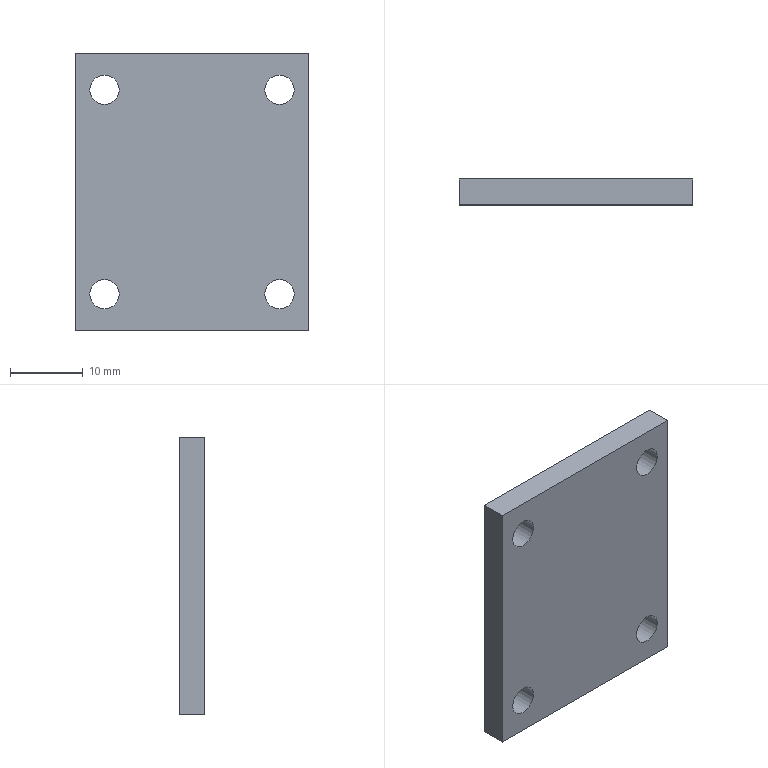Component | NX | OUTER_COVER_PLATE | 1 solid | 10 faces | box 32 x 3.5 x 38 mm | volume 4078 mm3 | plane 6 | cylinder 4 | commonest cylinder face diameters 4.024 x4
STEP:
#1=CARTESIAN_POINT('',(0.,0.,0.));
#2=DIRECTION('',(0.,0.,1.));
#3=DIRECTION('',(1.,0.,0.));
#4=AXIS2_PLACEMENT_3D('',#1,#2,#3);
#5=CARTESIAN_POINT('',(16.,29.,162.5));
#6=VERTEX_POINT('',#5);
#7=CARTESIAN_POINT('',(-16.,29.,162.5));
#8=VERTEX_POINT('',#7);
#9=CARTESIAN_POINT('',(16.,29.,162.5));
#10=DIRECTION('',(-1.,0.,0.));
#11=VECTOR('',#10,1.);
#12=LINE('',#9,#11);
#13=CARTESIAN_POINT('',(16.,32.5,162.5));
#14=DIRECTION('',(0.,0.,1.));
#15=DIRECTION('',(0.,-1.,0.));
#16=AXIS2_PLACEMENT_3D('',#13,#14,#15);
#17=PLANE('',#16);
#18=CARTESIAN_POINT('',(3.5,0.));
#19=DIRECTION('',(0.,-1.));
#20=VECTOR('',#19,1.);
#21=LINE('',#18,#20);
#22=(GEOMETRIC_REPRESENTATION_CONTEXT(2)PARAMETRIC_REPRESENTATION_CONTEXT()REPRESENTATION_CONTEXT('',''));
#23=DEFINITIONAL_REPRESENTATION('',(#21),#22);
#24=PCURVE('',#17,#23);
#25=CARTESIAN_POINT('',(12.,29.,129.5));
#26=DIRECTION('',(0.,1.,0.));
#27=DIRECTION('',(1.,0.,0.));
#28=AXIS2_PLACEMENT_3D('',#25,#26,#27);
#29=PLANE('',#28);
#30=CARTESIAN_POINT('',(4.,-33.));
#31=DIRECTION('',(-1.,0.));
#32=VECTOR('',#31,1.);
#33=LINE('',#30,#32);
#34=(GEOMETRIC_REPRESENTATION_CONTEXT(2)PARAMETRIC_REPRESENTATION_CONTEXT()REPRESENTATION_CONTEXT('',''));
#35=DEFINITIONAL_REPRESENTATION('',(#33),#34);
#36=PCURVE('',#29,#35);
#37=SURFACE_CURVE('',#12,(#24,#36),.PCURVE_S1.);
#38=EDGE_CURVE('',#6,#8,#37,.T.);
#39=ORIENTED_EDGE('',*,*,#38,.F.);
#40=CARTESIAN_POINT('',(16.,32.5,162.5));
#41=VERTEX_POINT('',#40);
#42=CARTESIAN_POINT('',(16.,32.5,162.5));
#43=DIRECTION('',(0.,-1.,0.));
#44=VECTOR('',#43,1.);
#45=LINE('',#42,#44);
#46=CARTESIAN_POINT('',(0.,0.));
#47=DIRECTION('',(1.,0.));
#48=VECTOR('',#47,1.);
#49=LINE('',#46,#48);
#50=(GEOMETRIC_REPRESENTATION_CONTEXT(2)PARAMETRIC_REPRESENTATION_CONTEXT()REPRESENTATION_CONTEXT('',''));
#51=DEFINITIONAL_REPRESENTATION('',(#49),#50);
#52=PCURVE('',#17,#51);
#53=CARTESIAN_POINT('',(16.,32.5,124.5));
#54=DIRECTION('',(1.,0.,0.));
#55=DIRECTION('',(0.,-1.,0.));
#56=AXIS2_PLACEMENT_3D('',#53,#54,#55);
#57=PLANE('',#56);
#58=CARTESIAN_POINT('',(0.,-38.));
#59=DIRECTION('',(1.,0.));
#60=VECTOR('',#59,1.);
#61=LINE('',#58,#60);
#62=(GEOMETRIC_REPRESENTATION_CONTEXT(2)PARAMETRIC_REPRESENTATION_CONTEXT()REPRESENTATION_CONTEXT('',''));
#63=DEFINITIONAL_REPRESENTATION('',(#61),#62);
#64=PCURVE('',#57,#63);
#65=SURFACE_CURVE('',#45,(#52,#64),.PCURVE_S1.);
#66=EDGE_CURVE('',#41,#6,#65,.T.);
#67=ORIENTED_EDGE('',*,*,#66,.F.);
#68=CARTESIAN_POINT('',(-16.,32.5,162.5));
#69=VERTEX_POINT('',#68);
#70=CARTESIAN_POINT('',(16.,32.5,162.5));
#71=DIRECTION('',(-1.,0.,0.));
#72=VECTOR('',#71,1.);
#73=LINE('',#70,#72);
#74=CARTESIAN_POINT('',(0.,0.));
#75=DIRECTION('',(0.,-1.));
#76=VECTOR('',#75,1.);
#77=LINE('',#74,#76);
#78=(GEOMETRIC_REPRESENTATION_CONTEXT(2)PARAMETRIC_REPRESENTATION_CONTEXT()REPRESENTATION_CONTEXT('',''));
#79=DEFINITIONAL_REPRESENTATION('',(#77),#78);
#80=PCURVE('',#17,#79);
#81=CARTESIAN_POINT('',(12.,32.5,129.5));
#82=DIRECTION('',(0.,1.,0.));
#83=DIRECTION('',(1.,0.,0.));
#84=AXIS2_PLACEMENT_3D('',#81,#82,#83);
#85=PLANE('',#84);
#86=CARTESIAN_POINT('',(4.,-33.));
#87=DIRECTION('',(-1.,0.));
#88=VECTOR('',#87,1.);
#89=LINE('',#86,#88);
#90=(GEOMETRIC_REPRESENTATION_CONTEXT(2)PARAMETRIC_REPRESENTATION_CONTEXT()REPRESENTATION_CONTEXT('',''));
#91=DEFINITIONAL_REPRESENTATION('',(#89),#90);
#92=PCURVE('',#85,#91);
#93=SURFACE_CURVE('',#73,(#80,#92),.PCURVE_S1.);
#94=EDGE_CURVE('',#41,#69,#93,.T.);
#95=ORIENTED_EDGE('',*,*,#94,.T.);
#96=CARTESIAN_POINT('',(-16.,32.5,162.5));
#97=DIRECTION('',(0.,-1.,0.));
#98=VECTOR('',#97,1.);
#99=LINE('',#96,#98);
#100=CARTESIAN_POINT('',(0.,-32.));
#101=DIRECTION('',(1.,0.));
#102=VECTOR('',#101,1.);
#103=LINE('',#100,#102);
#104=(GEOMETRIC_REPRESENTATION_CONTEXT(2)PARAMETRIC_REPRESENTATION_CONTEXT()REPRESENTATION_CONTEXT('',''));
#105=DEFINITIONAL_REPRESENTATION('',(#103),#104);
#106=PCURVE('',#17,#105);
#107=CARTESIAN_POINT('',(-16.,32.5,162.5));
#108=DIRECTION('',(-1.,0.,0.));
#109=DIRECTION('',(0.,1.,0.));
#110=AXIS2_PLACEMENT_3D('',#107,#108,#109);
#111=PLANE('',#110);
#112=CARTESIAN_POINT('',(0.,0.));
#113=DIRECTION('',(-1.,0.));
#114=VECTOR('',#113,1.);
#115=LINE('',#112,#114);
#116=(GEOMETRIC_REPRESENTATION_CONTEXT(2)PARAMETRIC_REPRESENTATION_CONTEXT()REPRESENTATION_CONTEXT('',''));
#117=DEFINITIONAL_REPRESENTATION('',(#115),#116);
#118=PCURVE('',#111,#117);
#119=SURFACE_CURVE('',#99,(#106,#118),.PCURVE_S1.);
#120=EDGE_CURVE('',#69,#8,#119,.T.);
#121=ORIENTED_EDGE('',*,*,#120,.T.);
#122=EDGE_LOOP('',(#39,#67,#95,#121));
#123=FACE_BOUND('',#122,.T.);
#124=ADVANCED_FACE('',(#123),#17,.T.);
#125=CARTESIAN_POINT('',(-16.,29.,124.5));
#126=VERTEX_POINT('',#125);
#127=CARTESIAN_POINT('',(-16.,29.,162.5));
#128=DIRECTION('',(0.,0.,-1.));
#129=VECTOR('',#128,1.);
#130=LINE('',#127,#129);
#131=CARTESIAN_POINT('',(-3.5,0.));
#132=DIRECTION('',(0.,1.));
#133=VECTOR('',#132,1.);
#134=LINE('',#131,#133);
#135=(GEOMETRIC_REPRESENTATION_CONTEXT(2)PARAMETRIC_REPRESENTATION_CONTEXT()REPRESENTATION_CONTEXT('',''));
#136=DEFINITIONAL_REPRESENTATION('',(#134),#135);
#137=PCURVE('',#111,#136);
#138=CARTESIAN_POINT('',(-28.,-33.));
#139=DIRECTION('',(0.,1.));
#140=VECTOR('',#139,1.);
#141=LINE('',#138,#140);
#142=(GEOMETRIC_REPRESENTATION_CONTEXT(2)PARAMETRIC_REPRESENTATION_CONTEXT()REPRESENTATION_CONTEXT('',''));
#143=DEFINITIONAL_REPRESENTATION('',(#141),#142);
#144=PCURVE('',#29,#143);
#145=SURFACE_CURVE('',#130,(#137,#144),.PCURVE_S1.);
#146=EDGE_CURVE('',#8,#126,#145,.T.);
#147=ORIENTED_EDGE('',*,*,#146,.F.);
#148=ORIENTED_EDGE('',*,*,#120,.F.);
#149=CARTESIAN_POINT('',(-16.,32.5,124.5));
#150=VERTEX_POINT('',#149);
#151=CARTESIAN_POINT('',(-16.,32.5,162.5));
#152=DIRECTION('',(0.,0.,-1.));
#153=VECTOR('',#152,1.);
#154=LINE('',#151,#153);
#155=CARTESIAN_POINT('',(0.,0.));
#156=DIRECTION('',(0.,1.));
#157=VECTOR('',#156,1.);
#158=LINE('',#155,#157);
#159=(GEOMETRIC_REPRESENTATION_CONTEXT(2)PARAMETRIC_REPRESENTATION_CONTEXT()REPRESENTATION_CONTEXT('',''));
#160=DEFINITIONAL_REPRESENTATION('',(#158),#159);
#161=PCURVE('',#111,#160);
#162=CARTESIAN_POINT('',(-28.,-33.));
#163=DIRECTION('',(0.,1.));
#164=VECTOR('',#163,1.);
#165=LINE('',#162,#164);
#166=(GEOMETRIC_REPRESENTATION_CONTEXT(2)PARAMETRIC_REPRESENTATION_CONTEXT()REPRESENTATION_CONTEXT('',''));
#167=DEFINITIONAL_REPRESENTATION('',(#165),#166);
#168=PCURVE('',#85,#167);
#169=SURFACE_CURVE('',#154,(#161,#168),.PCURVE_S1.);
#170=EDGE_CURVE('',#69,#150,#169,.T.);
#171=ORIENTED_EDGE('',*,*,#170,.T.);
#172=CARTESIAN_POINT('',(-16.,32.5,124.5));
#173=DIRECTION('',(0.,-1.,0.));
#174=VECTOR('',#173,1.);
#175=LINE('',#172,#174);
#176=CARTESIAN_POINT('',(0.,38.));
#177=DIRECTION('',(-1.,0.));
#178=VECTOR('',#177,1.);
#179=LINE('',#176,#178);
#180=(GEOMETRIC_REPRESENTATION_CONTEXT(2)PARAMETRIC_REPRESENTATION_CONTEXT()REPRESENTATION_CONTEXT('',''));
#181=DEFINITIONAL_REPRESENTATION('',(#179),#180);
#182=PCURVE('',#111,#181);
#183=CARTESIAN_POINT('',(-16.,32.5,124.5));
#184=DIRECTION('',(0.,0.,-1.));
#185=DIRECTION('',(0.,1.,0.));
#186=AXIS2_PLACEMENT_3D('',#183,#184,#185);
#187=PLANE('',#186);
#188=CARTESIAN_POINT('',(0.,0.));
#189=DIRECTION('',(-1.,0.));
#190=VECTOR('',#189,1.);
#191=LINE('',#188,#190);
#192=(GEOMETRIC_REPRESENTATION_CONTEXT(2)PARAMETRIC_REPRESENTATION_CONTEXT()REPRESENTATION_CONTEXT('',''));
#193=DEFINITIONAL_REPRESENTATION('',(#191),#192);
#194=PCURVE('',#187,#193);
#195=SURFACE_CURVE('',#175,(#182,#194),.PCURVE_S1.);
#196=EDGE_CURVE('',#150,#126,#195,.T.);
#197=ORIENTED_EDGE('',*,*,#196,.T.);
#198=EDGE_LOOP('',(#147,#148,#171,#197));
#199=FACE_BOUND('',#198,.T.);
#200=ADVANCED_FACE('',(#199),#111,.T.);
#201=CARTESIAN_POINT('',(16.,29.,124.5));
#202=VERTEX_POINT('',#201);
#203=CARTESIAN_POINT('',(-16.,29.,124.5));
#204=DIRECTION('',(1.,0.,0.));
#205=VECTOR('',#204,1.);
#206=LINE('',#203,#205);
#207=CARTESIAN_POINT('',(-3.5,0.));
#208=DIRECTION('',(0.,1.));
#209=VECTOR('',#208,1.);
#210=LINE('',#207,#209);
#211=(GEOMETRIC_REPRESENTATION_CONTEXT(2)PARAMETRIC_REPRESENTATION_CONTEXT()REPRESENTATION_CONTEXT('',''));
#212=DEFINITIONAL_REPRESENTATION('',(#210),#211);
#213=PCURVE('',#187,#212);
#214=CARTESIAN_POINT('',(-28.,5.));
#215=DIRECTION('',(1.,0.));
#216=VECTOR('',#215,1.);
#217=LINE('',#214,#216);
#218=(GEOMETRIC_REPRESENTATION_CONTEXT(2)PARAMETRIC_REPRESENTATION_CONTEXT()REPRESENTATION_CONTEXT('',''));
#219=DEFINITIONAL_REPRESENTATION('',(#217),#218);
#220=PCURVE('',#29,#219);
#221=SURFACE_CURVE('',#206,(#213,#220),.PCURVE_S1.);
#222=EDGE_CURVE('',#126,#202,#221,.T.);
#223=ORIENTED_EDGE('',*,*,#222,.F.);
#224=ORIENTED_EDGE('',*,*,#196,.F.);
#225=CARTESIAN_POINT('',(16.,32.5,124.5));
#226=VERTEX_POINT('',#225);
#227=CARTESIAN_POINT('',(-16.,32.5,124.5));
#228=DIRECTION('',(1.,0.,0.));
#229=VECTOR('',#228,1.);
#230=LINE('',#227,#229);
#231=CARTESIAN_POINT('',(0.,0.));
#232=DIRECTION('',(0.,1.));
#233=VECTOR('',#232,1.);
#234=LINE('',#231,#233);
#235=(GEOMETRIC_REPRESENTATION_CONTEXT(2)PARAMETRIC_REPRESENTATION_CONTEXT()REPRESENTATION_CONTEXT('',''));
#236=DEFINITIONAL_REPRESENTATION('',(#234),#235);
#237=PCURVE('',#187,#236);
#238=CARTESIAN_POINT('',(-28.,5.));
#239=DIRECTION('',(1.,0.));
#240=VECTOR('',#239,1.);
#241=LINE('',#238,#240);
#242=(GEOMETRIC_REPRESENTATION_CONTEXT(2)PARAMETRIC_REPRESENTATION_CONTEXT()REPRESENTATION_CONTEXT('',''));
#243=DEFINITIONAL_REPRESENTATION('',(#241),#242);
#244=PCURVE('',#85,#243);
#245=SURFACE_CURVE('',#230,(#237,#244),.PCURVE_S1.);
#246=EDGE_CURVE('',#150,#226,#245,.T.);
#247=ORIENTED_EDGE('',*,*,#246,.T.);
#248=CARTESIAN_POINT('',(16.,32.5,124.5));
#249=DIRECTION('',(0.,-1.,0.));
#250=VECTOR('',#249,1.);
#251=LINE('',#248,#250);
#252=CARTESIAN_POINT('',(0.,32.));
#253=DIRECTION('',(-1.,0.));
#254=VECTOR('',#253,1.);
#255=LINE('',#252,#254);
#256=(GEOMETRIC_REPRESENTATION_CONTEXT(2)PARAMETRIC_REPRESENTATION_CONTEXT()REPRESENTATION_CONTEXT('',''));
#257=DEFINITIONAL_REPRESENTATION('',(#255),#256);
#258=PCURVE('',#187,#257);
#259=CARTESIAN_POINT('',(0.,0.));
#260=DIRECTION('',(1.,0.));
#261=VECTOR('',#260,1.);
#262=LINE('',#259,#261);
#263=(GEOMETRIC_REPRESENTATION_CONTEXT(2)PARAMETRIC_REPRESENTATION_CONTEXT()REPRESENTATION_CONTEXT('',''));
#264=DEFINITIONAL_REPRESENTATION('',(#262),#263);
#265=PCURVE('',#57,#264);
#266=SURFACE_CURVE('',#251,(#258,#265),.PCURVE_S1.);
#267=EDGE_CURVE('',#226,#202,#266,.T.);
#268=ORIENTED_EDGE('',*,*,#267,.T.);
#269=EDGE_LOOP('',(#223,#224,#247,#268));
#270=FACE_BOUND('',#269,.T.);
#271=ADVANCED_FACE('',(#270),#187,.T.);
#272=CARTESIAN_POINT('',(16.,29.,124.5));
#273=DIRECTION('',(0.,0.,1.));
#274=VECTOR('',#273,1.);
#275=LINE('',#272,#274);
#276=CARTESIAN_POINT('',(3.5,0.));
#277=DIRECTION('',(0.,-1.));
#278=VECTOR('',#277,1.);
#279=LINE('',#276,#278);
#280=(GEOMETRIC_REPRESENTATION_CONTEXT(2)PARAMETRIC_REPRESENTATION_CONTEXT()REPRESENTATION_CONTEXT('',''));
#281=DEFINITIONAL_REPRESENTATION('',(#279),#280);
#282=PCURVE('',#57,#281);
#283=CARTESIAN_POINT('',(4.,5.));
#284=DIRECTION('',(0.,-1.));
#285=VECTOR('',#284,1.);
#286=LINE('',#283,#285);
#287=(GEOMETRIC_REPRESENTATION_CONTEXT(2)PARAMETRIC_REPRESENTATION_CONTEXT()REPRESENTATION_CONTEXT('',''));
#288=DEFINITIONAL_REPRESENTATION('',(#286),#287);
#289=PCURVE('',#29,#288);
#290=SURFACE_CURVE('',#275,(#282,#289),.PCURVE_S1.);
#291=EDGE_CURVE('',#202,#6,#290,.T.);
#292=ORIENTED_EDGE('',*,*,#291,.F.);
#293=ORIENTED_EDGE('',*,*,#267,.F.);
#294=CARTESIAN_POINT('',(16.,32.5,124.5));
#295=DIRECTION('',(0.,0.,1.));
#296=VECTOR('',#295,1.);
#297=LINE('',#294,#296);
#298=CARTESIAN_POINT('',(0.,0.));
#299=DIRECTION('',(0.,-1.));
#300=VECTOR('',#299,1.);
#301=LINE('',#298,#300);
#302=(GEOMETRIC_REPRESENTATION_CONTEXT(2)PARAMETRIC_REPRESENTATION_CONTEXT()REPRESENTATION_CONTEXT('',''));
#303=DEFINITIONAL_REPRESENTATION('',(#301),#302);
#304=PCURVE('',#57,#303);
#305=CARTESIAN_POINT('',(4.,5.));
#306=DIRECTION('',(0.,-1.));
#307=VECTOR('',#306,1.);
#308=LINE('',#305,#307);
#309=(GEOMETRIC_REPRESENTATION_CONTEXT(2)PARAMETRIC_REPRESENTATION_CONTEXT()REPRESENTATION_CONTEXT('',''));
#310=DEFINITIONAL_REPRESENTATION('',(#308),#309);
#311=PCURVE('',#85,#310);
#312=SURFACE_CURVE('',#297,(#304,#311),.PCURVE_S1.);
#313=EDGE_CURVE('',#226,#41,#312,.T.);
#314=ORIENTED_EDGE('',*,*,#313,.T.);
#315=ORIENTED_EDGE('',*,*,#66,.T.);
#316=EDGE_LOOP('',(#292,#293,#314,#315));
#317=FACE_BOUND('',#316,.T.);
#318=ADVANCED_FACE('',(#317),#57,.T.);
#319=CARTESIAN_POINT('',(14.012,32.5,157.5));
#320=VERTEX_POINT('',#319);
#321=CARTESIAN_POINT('',(12.,32.5,157.5));
#322=DIRECTION('',(0.,1.,0.));
#323=DIRECTION('',(1.,0.,0.));
#324=AXIS2_PLACEMENT_3D('',#321,#322,#323);
#325=CIRCLE('',#324,2.012);
#326=CARTESIAN_POINT('',(0.,-28.));
#327=DIRECTION('',(1.,0.));
#328=AXIS2_PLACEMENT_2D('',#326,#327);
#329=CIRCLE('',#328,2.012);
#330=(GEOMETRIC_REPRESENTATION_CONTEXT(2)PARAMETRIC_REPRESENTATION_CONTEXT()REPRESENTATION_CONTEXT('',''));
#331=DEFINITIONAL_REPRESENTATION('',(#329),#330);
#332=PCURVE('',#85,#331);
#333=CARTESIAN_POINT('',(12.,28.9,157.5));
#334=DIRECTION('',(-0.,1.,0.));
#335=DIRECTION('',(1.,0.,0.));
#336=AXIS2_PLACEMENT_3D('',#333,#334,#335);
#337=CYLINDRICAL_SURFACE('',#336,2.012);
#338=CARTESIAN_POINT('',(0.,3.6));
#339=DIRECTION('',(1.,0.));
#340=VECTOR('',#339,1.);
#341=LINE('',#338,#340);
#342=(GEOMETRIC_REPRESENTATION_CONTEXT(2)PARAMETRIC_REPRESENTATION_CONTEXT()REPRESENTATION_CONTEXT('',''));
#343=DEFINITIONAL_REPRESENTATION('',(#341),#342);
#344=PCURVE('',#337,#343);
#345=SURFACE_CURVE('',#325,(#332,#344),.PCURVE_S1.);
#346=EDGE_CURVE('',#320,#320,#345,.T.);
#347=ORIENTED_EDGE('',*,*,#346,.F.);
#348=EDGE_LOOP('',(#347));
#349=FACE_BOUND('',#348,.T.);
#350=CARTESIAN_POINT('',(-9.988,32.5,157.5));
#351=VERTEX_POINT('',#350);
#352=CARTESIAN_POINT('',(-12.,32.5,157.5));
#353=DIRECTION('',(0.,1.,0.));
#354=DIRECTION('',(1.,0.,0.));
#355=AXIS2_PLACEMENT_3D('',#352,#353,#354);
#356=CIRCLE('',#355,2.012);
#357=CARTESIAN_POINT('',(-24.,-28.));
#358=DIRECTION('',(1.,0.));
#359=AXIS2_PLACEMENT_2D('',#357,#358);
#360=CIRCLE('',#359,2.012);
#361=(GEOMETRIC_REPRESENTATION_CONTEXT(2)PARAMETRIC_REPRESENTATION_CONTEXT()REPRESENTATION_CONTEXT('',''));
#362=DEFINITIONAL_REPRESENTATION('',(#360),#361);
#363=PCURVE('',#85,#362);
#364=CARTESIAN_POINT('',(-12.,28.9,157.5));
#365=DIRECTION('',(-0.,1.,0.));
#366=DIRECTION('',(1.,0.,0.));
#367=AXIS2_PLACEMENT_3D('',#364,#365,#366);
#368=CYLINDRICAL_SURFACE('',#367,2.012);
#369=CARTESIAN_POINT('',(0.,3.6));
#370=DIRECTION('',(1.,0.));
#371=VECTOR('',#370,1.);
#372=LINE('',#369,#371);
#373=(GEOMETRIC_REPRESENTATION_CONTEXT(2)PARAMETRIC_REPRESENTATION_CONTEXT()REPRESENTATION_CONTEXT('',''));
#374=DEFINITIONAL_REPRESENTATION('',(#372),#373);
#375=PCURVE('',#368,#374);
#376=SURFACE_CURVE('',#356,(#363,#375),.PCURVE_S1.);
#377=EDGE_CURVE('',#351,#351,#376,.T.);
#378=ORIENTED_EDGE('',*,*,#377,.F.);
#379=EDGE_LOOP('',(#378));
#380=FACE_BOUND('',#379,.T.);
#381=CARTESIAN_POINT('',(14.012,32.5,129.5));
#382=VERTEX_POINT('',#381);
#383=CARTESIAN_POINT('',(12.,32.5,129.5));
#384=DIRECTION('',(0.,1.,0.));
#385=DIRECTION('',(1.,0.,0.));
#386=AXIS2_PLACEMENT_3D('',#383,#384,#385);
#387=CIRCLE('',#386,2.012);
#388=CARTESIAN_POINT('',(0.,0.));
#389=DIRECTION('',(1.,0.));
#390=AXIS2_PLACEMENT_2D('',#388,#389);
#391=CIRCLE('',#390,2.012);
#392=(GEOMETRIC_REPRESENTATION_CONTEXT(2)PARAMETRIC_REPRESENTATION_CONTEXT()REPRESENTATION_CONTEXT('',''));
#393=DEFINITIONAL_REPRESENTATION('',(#391),#392);
#394=PCURVE('',#85,#393);
#395=CARTESIAN_POINT('',(12.,28.9,129.5));
#396=DIRECTION('',(-0.,1.,0.));
#397=DIRECTION('',(1.,0.,0.));
#398=AXIS2_PLACEMENT_3D('',#395,#396,#397);
#399=CYLINDRICAL_SURFACE('',#398,2.012);
#400=CARTESIAN_POINT('',(0.,3.6));
#401=DIRECTION('',(1.,0.));
#402=VECTOR('',#401,1.);
#403=LINE('',#400,#402);
#404=(GEOMETRIC_REPRESENTATION_CONTEXT(2)PARAMETRIC_REPRESENTATION_CONTEXT()REPRESENTATION_CONTEXT('',''));
#405=DEFINITIONAL_REPRESENTATION('',(#403),#404);
#406=PCURVE('',#399,#405);
#407=SURFACE_CURVE('',#387,(#394,#406),.PCURVE_S1.);
#408=EDGE_CURVE('',#382,#382,#407,.T.);
#409=ORIENTED_EDGE('',*,*,#408,.F.);
#410=EDGE_LOOP('',(#409));
#411=FACE_BOUND('',#410,.T.);
#412=CARTESIAN_POINT('',(-9.988,32.5,129.5));
#413=VERTEX_POINT('',#412);
#414=CARTESIAN_POINT('',(-12.,32.5,129.5));
#415=DIRECTION('',(0.,1.,0.));
#416=DIRECTION('',(1.,0.,0.));
#417=AXIS2_PLACEMENT_3D('',#414,#415,#416);
#418=CIRCLE('',#417,2.012);
#419=CARTESIAN_POINT('',(-24.,0.));
#420=DIRECTION('',(1.,0.));
#421=AXIS2_PLACEMENT_2D('',#419,#420);
#422=CIRCLE('',#421,2.012);
#423=(GEOMETRIC_REPRESENTATION_CONTEXT(2)PARAMETRIC_REPRESENTATION_CONTEXT()REPRESENTATION_CONTEXT('',''));
#424=DEFINITIONAL_REPRESENTATION('',(#422),#423);
#425=PCURVE('',#85,#424);
#426=CARTESIAN_POINT('',(-12.,28.9,129.5));
#427=DIRECTION('',(-0.,1.,0.));
#428=DIRECTION('',(1.,0.,0.));
#429=AXIS2_PLACEMENT_3D('',#426,#427,#428);
#430=CYLINDRICAL_SURFACE('',#429,2.012);
#431=CARTESIAN_POINT('',(0.,3.6));
#432=DIRECTION('',(1.,0.));
#433=VECTOR('',#432,1.);
#434=LINE('',#431,#433);
#435=(GEOMETRIC_REPRESENTATION_CONTEXT(2)PARAMETRIC_REPRESENTATION_CONTEXT()REPRESENTATION_CONTEXT('',''));
#436=DEFINITIONAL_REPRESENTATION('',(#434),#435);
#437=PCURVE('',#430,#436);
#438=SURFACE_CURVE('',#418,(#425,#437),.PCURVE_S1.);
#439=EDGE_CURVE('',#413,#413,#438,.T.);
#440=ORIENTED_EDGE('',*,*,#439,.F.);
#441=EDGE_LOOP('',(#440));
#442=FACE_BOUND('',#441,.T.);
#443=ORIENTED_EDGE('',*,*,#94,.F.);
#444=ORIENTED_EDGE('',*,*,#313,.F.);
#445=ORIENTED_EDGE('',*,*,#246,.F.);
#446=ORIENTED_EDGE('',*,*,#170,.F.);
#447=EDGE_LOOP('',(#443,#444,#445,#446));
#448=FACE_BOUND('',#447,.T.);
#449=ADVANCED_FACE('',(#349,#380,#411,#442,#448),#85,.T.);
#450=CARTESIAN_POINT('',(14.012,29.,157.5));
#451=VERTEX_POINT('',#450);
#452=CARTESIAN_POINT('',(12.,29.,157.5));
#453=DIRECTION('',(0.,1.,0.));
#454=DIRECTION('',(1.,0.,0.));
#455=AXIS2_PLACEMENT_3D('',#452,#453,#454);
#456=CIRCLE('',#455,2.012);
#457=CARTESIAN_POINT('',(0.,-28.));
#458=DIRECTION('',(1.,0.));
#459=AXIS2_PLACEMENT_2D('',#457,#458);
#460=CIRCLE('',#459,2.012);
#461=(GEOMETRIC_REPRESENTATION_CONTEXT(2)PARAMETRIC_REPRESENTATION_CONTEXT()REPRESENTATION_CONTEXT('',''));
#462=DEFINITIONAL_REPRESENTATION('',(#460),#461);
#463=PCURVE('',#29,#462);
#464=CARTESIAN_POINT('',(0.,0.1));
#465=DIRECTION('',(1.,0.));
#466=VECTOR('',#465,1.);
#467=LINE('',#464,#466);
#468=(GEOMETRIC_REPRESENTATION_CONTEXT(2)PARAMETRIC_REPRESENTATION_CONTEXT()REPRESENTATION_CONTEXT('',''));
#469=DEFINITIONAL_REPRESENTATION('',(#467),#468);
#470=PCURVE('',#337,#469);
#471=SURFACE_CURVE('',#456,(#463,#470),.PCURVE_S1.);
#472=EDGE_CURVE('',#451,#451,#471,.T.);
#473=ORIENTED_EDGE('',*,*,#472,.T.);
#474=EDGE_LOOP('',(#473));
#475=FACE_BOUND('',#474,.T.);
#476=CARTESIAN_POINT('',(-9.988,29.,157.5));
#477=VERTEX_POINT('',#476);
#478=CARTESIAN_POINT('',(-12.,29.,157.5));
#479=DIRECTION('',(0.,1.,0.));
#480=DIRECTION('',(1.,0.,0.));
#481=AXIS2_PLACEMENT_3D('',#478,#479,#480);
#482=CIRCLE('',#481,2.012);
#483=CARTESIAN_POINT('',(-24.,-28.));
#484=DIRECTION('',(1.,0.));
#485=AXIS2_PLACEMENT_2D('',#483,#484);
#486=CIRCLE('',#485,2.012);
#487=(GEOMETRIC_REPRESENTATION_CONTEXT(2)PARAMETRIC_REPRESENTATION_CONTEXT()REPRESENTATION_CONTEXT('',''));
#488=DEFINITIONAL_REPRESENTATION('',(#486),#487);
#489=PCURVE('',#29,#488);
#490=CARTESIAN_POINT('',(0.,0.1));
#491=DIRECTION('',(1.,0.));
#492=VECTOR('',#491,1.);
#493=LINE('',#490,#492);
#494=(GEOMETRIC_REPRESENTATION_CONTEXT(2)PARAMETRIC_REPRESENTATION_CONTEXT()REPRESENTATION_CONTEXT('',''));
#495=DEFINITIONAL_REPRESENTATION('',(#493),#494);
#496=PCURVE('',#368,#495);
#497=SURFACE_CURVE('',#482,(#489,#496),.PCURVE_S1.);
#498=EDGE_CURVE('',#477,#477,#497,.T.);
#499=ORIENTED_EDGE('',*,*,#498,.T.);
#500=EDGE_LOOP('',(#499));
#501=FACE_BOUND('',#500,.T.);
#502=CARTESIAN_POINT('',(14.012,29.,129.5));
#503=VERTEX_POINT('',#502);
#504=CARTESIAN_POINT('',(12.,29.,129.5));
#505=DIRECTION('',(0.,1.,0.));
#506=DIRECTION('',(1.,0.,0.));
#507=AXIS2_PLACEMENT_3D('',#504,#505,#506);
#508=CIRCLE('',#507,2.012);
#509=CARTESIAN_POINT('',(0.,0.));
#510=DIRECTION('',(1.,0.));
#511=AXIS2_PLACEMENT_2D('',#509,#510);
#512=CIRCLE('',#511,2.012);
#513=(GEOMETRIC_REPRESENTATION_CONTEXT(2)PARAMETRIC_REPRESENTATION_CONTEXT()REPRESENTATION_CONTEXT('',''));
#514=DEFINITIONAL_REPRESENTATION('',(#512),#513);
#515=PCURVE('',#29,#514);
#516=CARTESIAN_POINT('',(0.,0.1));
#517=DIRECTION('',(1.,0.));
#518=VECTOR('',#517,1.);
#519=LINE('',#516,#518);
#520=(GEOMETRIC_REPRESENTATION_CONTEXT(2)PARAMETRIC_REPRESENTATION_CONTEXT()REPRESENTATION_CONTEXT('',''));
#521=DEFINITIONAL_REPRESENTATION('',(#519),#520);
#522=PCURVE('',#399,#521);
#523=SURFACE_CURVE('',#508,(#515,#522),.PCURVE_S1.);
#524=EDGE_CURVE('',#503,#503,#523,.T.);
#525=ORIENTED_EDGE('',*,*,#524,.T.);
#526=EDGE_LOOP('',(#525));
#527=FACE_BOUND('',#526,.T.);
#528=CARTESIAN_POINT('',(-9.988,29.,129.5));
#529=VERTEX_POINT('',#528);
#530=CARTESIAN_POINT('',(-12.,29.,129.5));
#531=DIRECTION('',(0.,1.,0.));
#532=DIRECTION('',(1.,0.,0.));
#533=AXIS2_PLACEMENT_3D('',#530,#531,#532);
#534=CIRCLE('',#533,2.012);
#535=CARTESIAN_POINT('',(-24.,0.));
#536=DIRECTION('',(1.,0.));
#537=AXIS2_PLACEMENT_2D('',#535,#536);
#538=CIRCLE('',#537,2.012);
#539=(GEOMETRIC_REPRESENTATION_CONTEXT(2)PARAMETRIC_REPRESENTATION_CONTEXT()REPRESENTATION_CONTEXT('',''));
#540=DEFINITIONAL_REPRESENTATION('',(#538),#539);
#541=PCURVE('',#29,#540);
#542=CARTESIAN_POINT('',(0.,0.1));
#543=DIRECTION('',(1.,0.));
#544=VECTOR('',#543,1.);
#545=LINE('',#542,#544);
#546=(GEOMETRIC_REPRESENTATION_CONTEXT(2)PARAMETRIC_REPRESENTATION_CONTEXT()REPRESENTATION_CONTEXT('',''));
#547=DEFINITIONAL_REPRESENTATION('',(#545),#546);
#548=PCURVE('',#430,#547);
#549=SURFACE_CURVE('',#534,(#541,#548),.PCURVE_S1.);
#550=EDGE_CURVE('',#529,#529,#549,.T.);
#551=ORIENTED_EDGE('',*,*,#550,.T.);
#552=EDGE_LOOP('',(#551));
#553=FACE_BOUND('',#552,.T.);
#554=ORIENTED_EDGE('',*,*,#38,.T.);
#555=ORIENTED_EDGE('',*,*,#146,.T.);
#556=ORIENTED_EDGE('',*,*,#222,.T.);
#557=ORIENTED_EDGE('',*,*,#291,.T.);
#558=EDGE_LOOP('',(#554,#555,#556,#557));
#559=FACE_BOUND('',#558,.T.);
#560=ADVANCED_FACE('',(#475,#501,#527,#553,#559),#29,.F.);
#561=ORIENTED_EDGE('',*,*,#439,.F.);
#562=CARTESIAN_POINT('',(-9.988,29.,129.5));
#563=CARTESIAN_POINT('',(-9.988,32.5,129.5));
#564=B_SPLINE_CURVE_WITH_KNOTS('',1,(#562,#563),.UNSPECIFIED.,.F.,.F.,(2,2),(0.1,3.6),.PIECEWISE_BEZIER_KNOTS.);
#565=CARTESIAN_POINT('',(0.,0.));
#566=DIRECTION('',(0.,1.));
#567=VECTOR('',#566,1.);
#568=LINE('',#565,#567);
#569=(GEOMETRIC_REPRESENTATION_CONTEXT(2)PARAMETRIC_REPRESENTATION_CONTEXT()REPRESENTATION_CONTEXT('',''));
#570=DEFINITIONAL_REPRESENTATION('',(#568),#569);
#571=PCURVE('',#430,#570);
#572=CARTESIAN_POINT('',(6.283,0.));
#573=DIRECTION('',(0.,1.));
#574=VECTOR('',#573,1.);
#575=LINE('',#572,#574);
#576=(GEOMETRIC_REPRESENTATION_CONTEXT(2)PARAMETRIC_REPRESENTATION_CONTEXT()REPRESENTATION_CONTEXT('',''));
#577=DEFINITIONAL_REPRESENTATION('',(#575),#576);
#578=PCURVE('',#430,#577);
#579=SEAM_CURVE('',#564,(#571,#578),.PCURVE_S1.);
#580=EDGE_CURVE('',#529,#413,#579,.T.);
#581=ORIENTED_EDGE('',*,*,#580,.F.);
#582=ORIENTED_EDGE('',*,*,#550,.T.);
#583=ORIENTED_EDGE('',*,*,#580,.T.);
#584=EDGE_LOOP('',(#561,#581,#582,#583));
#585=FACE_BOUND('',#584,.F.);
#586=ADVANCED_FACE('',(#585),#430,.F.);
#587=ORIENTED_EDGE('',*,*,#408,.F.);
#588=CARTESIAN_POINT('',(14.012,29.,129.5));
#589=CARTESIAN_POINT('',(14.012,32.5,129.5));
#590=B_SPLINE_CURVE_WITH_KNOTS('',1,(#588,#589),.UNSPECIFIED.,.F.,.F.,(2,2),(0.1,3.6),.PIECEWISE_BEZIER_KNOTS.);
#591=CARTESIAN_POINT('',(0.,0.));
#592=DIRECTION('',(0.,1.));
#593=VECTOR('',#592,1.);
#594=LINE('',#591,#593);
#595=(GEOMETRIC_REPRESENTATION_CONTEXT(2)PARAMETRIC_REPRESENTATION_CONTEXT()REPRESENTATION_CONTEXT('',''));
#596=DEFINITIONAL_REPRESENTATION('',(#594),#595);
#597=PCURVE('',#399,#596);
#598=CARTESIAN_POINT('',(6.283,0.));
#599=DIRECTION('',(0.,1.));
#600=VECTOR('',#599,1.);
#601=LINE('',#598,#600);
#602=(GEOMETRIC_REPRESENTATION_CONTEXT(2)PARAMETRIC_REPRESENTATION_CONTEXT()REPRESENTATION_CONTEXT('',''));
#603=DEFINITIONAL_REPRESENTATION('',(#601),#602);
#604=PCURVE('',#399,#603);
#605=SEAM_CURVE('',#590,(#597,#604),.PCURVE_S1.);
#606=EDGE_CURVE('',#503,#382,#605,.T.);
#607=ORIENTED_EDGE('',*,*,#606,.F.);
#608=ORIENTED_EDGE('',*,*,#524,.T.);
#609=ORIENTED_EDGE('',*,*,#606,.T.);
#610=EDGE_LOOP('',(#587,#607,#608,#609));
#611=FACE_BOUND('',#610,.F.);
#612=ADVANCED_FACE('',(#611),#399,.F.);
#613=ORIENTED_EDGE('',*,*,#377,.F.);
#614=CARTESIAN_POINT('',(-9.988,29.,157.5));
#615=CARTESIAN_POINT('',(-9.988,32.5,157.5));
#616=B_SPLINE_CURVE_WITH_KNOTS('',1,(#614,#615),.UNSPECIFIED.,.F.,.F.,(2,2),(0.1,3.6),.PIECEWISE_BEZIER_KNOTS.);
#617=CARTESIAN_POINT('',(0.,0.));
#618=DIRECTION('',(0.,1.));
#619=VECTOR('',#618,1.);
#620=LINE('',#617,#619);
#621=(GEOMETRIC_REPRESENTATION_CONTEXT(2)PARAMETRIC_REPRESENTATION_CONTEXT()REPRESENTATION_CONTEXT('',''));
#622=DEFINITIONAL_REPRESENTATION('',(#620),#621);
#623=PCURVE('',#368,#622);
#624=CARTESIAN_POINT('',(6.283,0.));
#625=DIRECTION('',(0.,1.));
#626=VECTOR('',#625,1.);
#627=LINE('',#624,#626);
#628=(GEOMETRIC_REPRESENTATION_CONTEXT(2)PARAMETRIC_REPRESENTATION_CONTEXT()REPRESENTATION_CONTEXT('',''));
#629=DEFINITIONAL_REPRESENTATION('',(#627),#628);
#630=PCURVE('',#368,#629);
#631=SEAM_CURVE('',#616,(#623,#630),.PCURVE_S1.);
#632=EDGE_CURVE('',#477,#351,#631,.T.);
#633=ORIENTED_EDGE('',*,*,#632,.F.);
#634=ORIENTED_EDGE('',*,*,#498,.T.);
#635=ORIENTED_EDGE('',*,*,#632,.T.);
#636=EDGE_LOOP('',(#613,#633,#634,#635));
#637=FACE_BOUND('',#636,.F.);
#638=ADVANCED_FACE('',(#637),#368,.F.);
#639=ORIENTED_EDGE('',*,*,#346,.F.);
#640=CARTESIAN_POINT('',(14.012,29.,157.5));
#641=CARTESIAN_POINT('',(14.012,32.5,157.5));
#642=B_SPLINE_CURVE_WITH_KNOTS('',1,(#640,#641),.UNSPECIFIED.,.F.,.F.,(2,2),(0.1,3.6),.PIECEWISE_BEZIER_KNOTS.);
#643=CARTESIAN_POINT('',(0.,0.));
#644=DIRECTION('',(0.,1.));
#645=VECTOR('',#644,1.);
#646=LINE('',#643,#645);
#647=(GEOMETRIC_REPRESENTATION_CONTEXT(2)PARAMETRIC_REPRESENTATION_CONTEXT()REPRESENTATION_CONTEXT('',''));
#648=DEFINITIONAL_REPRESENTATION('',(#646),#647);
#649=PCURVE('',#337,#648);
#650=CARTESIAN_POINT('',(6.283,0.));
#651=DIRECTION('',(0.,1.));
#652=VECTOR('',#651,1.);
#653=LINE('',#650,#652);
#654=(GEOMETRIC_REPRESENTATION_CONTEXT(2)PARAMETRIC_REPRESENTATION_CONTEXT()REPRESENTATION_CONTEXT('',''));
#655=DEFINITIONAL_REPRESENTATION('',(#653),#654);
#656=PCURVE('',#337,#655);
#657=SEAM_CURVE('',#642,(#649,#656),.PCURVE_S1.);
#658=EDGE_CURVE('',#451,#320,#657,.T.);
#659=ORIENTED_EDGE('',*,*,#658,.F.);
#660=ORIENTED_EDGE('',*,*,#472,.T.);
#661=ORIENTED_EDGE('',*,*,#658,.T.);
#662=EDGE_LOOP('',(#639,#659,#660,#661));
#663=FACE_BOUND('',#662,.F.);
#664=ADVANCED_FACE('',(#663),#337,.F.);
#665=CLOSED_SHELL('',(#124,#200,#271,#318,#449,#560,#586,#612,#638,#664));
#666=MANIFOLD_SOLID_BREP('',#665);
#667=(LENGTH_UNIT()NAMED_UNIT(*)SI_UNIT(.MILLI.,.METRE.));
#668=UNCERTAINTY_MEASURE_WITH_UNIT(LENGTH_MEASURE(0.000005),#667,'','');
#669=(NAMED_UNIT(*)PLANE_ANGLE_UNIT()SI_UNIT($,.RADIAN.));
#670=(NAMED_UNIT(*)SI_UNIT($,.STERADIAN.)SOLID_ANGLE_UNIT());
#671=(GEOMETRIC_REPRESENTATION_CONTEXT(3)GLOBAL_UNCERTAINTY_ASSIGNED_CONTEXT((#668))GLOBAL_UNIT_ASSIGNED_CONTEXT((#667,#669,#670))REPRESENTATION_CONTEXT('',''));
#672=ADVANCED_BREP_SHAPE_REPRESENTATION('',(#4,#666),#671);